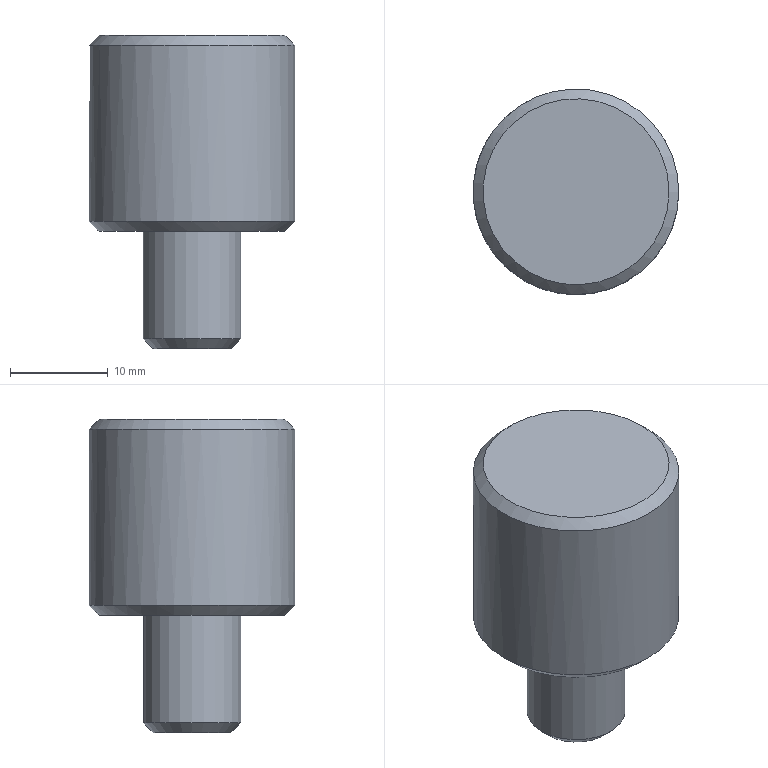Component | NX | FIXED_DOWEL_PIN | 1 solid | 8 faces | box 21 x 21 x 32 mm | volume 7791 mm3 | plane 3 | cone 3 | cylinder 2 | commonest cylinder face diameters 10 x1 21 x1
STEP:
#1=CARTESIAN_POINT('',(0.,0.,0.));
#2=DIRECTION('',(0.,0.,1.));
#3=DIRECTION('',(1.,0.,0.));
#4=AXIS2_PLACEMENT_3D('',#1,#2,#3);
#5=CARTESIAN_POINT('',(176.,0.,-79.));
#6=VERTEX_POINT('',#5);
#7=CARTESIAN_POINT('',(180.,0.,-79.));
#8=DIRECTION('',(0.,0.,-1.));
#9=DIRECTION('',(-1.,0.,0.));
#10=AXIS2_PLACEMENT_3D('',#7,#8,#9);
#11=CIRCLE('',#10,4.);
#12=CARTESIAN_POINT('',(180.,0.,-79.));
#13=DIRECTION('',(0.,0.,-1.));
#14=DIRECTION('',(-1.,0.,0.));
#15=AXIS2_PLACEMENT_3D('',#12,#13,#14);
#16=PLANE('',#15);
#17=CARTESIAN_POINT('',(0.,0.));
#18=DIRECTION('',(1.,0.));
#19=AXIS2_PLACEMENT_2D('',#17,#18);
#20=CIRCLE('',#19,4.);
#21=(GEOMETRIC_REPRESENTATION_CONTEXT(2)PARAMETRIC_REPRESENTATION_CONTEXT()REPRESENTATION_CONTEXT('',''));
#22=DEFINITIONAL_REPRESENTATION('',(#20),#21);
#23=PCURVE('',#16,#22);
#24=CARTESIAN_POINT('',(180.,0.,-78.));
#25=DIRECTION('',(0.,0.,1.));
#26=DIRECTION('',(1.,0.,0.));
#27=AXIS2_PLACEMENT_3D('',#24,#25,#26);
#28=CONICAL_SURFACE('',#27,5.,0.7854);
#29=CARTESIAN_POINT('',(9.425,-1.));
#30=DIRECTION('',(-1.,0.));
#31=VECTOR('',#30,1.);
#32=LINE('',#29,#31);
#33=(GEOMETRIC_REPRESENTATION_CONTEXT(2)PARAMETRIC_REPRESENTATION_CONTEXT()REPRESENTATION_CONTEXT('',''));
#34=DEFINITIONAL_REPRESENTATION('',(#32),#33);
#35=PCURVE('',#28,#34);
#36=SURFACE_CURVE('',#11,(#23,#35),.PCURVE_S1.);
#37=EDGE_CURVE('',#6,#6,#36,.T.);
#38=ORIENTED_EDGE('',*,*,#37,.T.);
#39=EDGE_LOOP('',(#38));
#40=FACE_BOUND('',#39,.T.);
#41=ADVANCED_FACE('',(#40),#16,.T.);
#42=CARTESIAN_POINT('',(175.,0.,-78.));
#43=VERTEX_POINT('',#42);
#44=CARTESIAN_POINT('',(180.,0.,-78.));
#45=DIRECTION('',(0.,0.,1.));
#46=DIRECTION('',(-1.,0.,0.));
#47=AXIS2_PLACEMENT_3D('',#44,#45,#46);
#48=CIRCLE('',#47,5.);
#49=CARTESIAN_POINT('',(180.,0.,-79.));
#50=DIRECTION('',(0.,0.,1.));
#51=DIRECTION('',(1.,0.,0.));
#52=AXIS2_PLACEMENT_3D('',#49,#50,#51);
#53=CYLINDRICAL_SURFACE('',#52,5.);
#54=CARTESIAN_POINT('',(3.142,1.));
#55=DIRECTION('',(1.,0.));
#56=VECTOR('',#55,1.);
#57=LINE('',#54,#56);
#58=(GEOMETRIC_REPRESENTATION_CONTEXT(2)PARAMETRIC_REPRESENTATION_CONTEXT()REPRESENTATION_CONTEXT('',''));
#59=DEFINITIONAL_REPRESENTATION('',(#57),#58);
#60=PCURVE('',#53,#59);
#61=CARTESIAN_POINT('',(3.142,0.));
#62=DIRECTION('',(1.,0.));
#63=VECTOR('',#62,1.);
#64=LINE('',#61,#63);
#65=(GEOMETRIC_REPRESENTATION_CONTEXT(2)PARAMETRIC_REPRESENTATION_CONTEXT()REPRESENTATION_CONTEXT('',''));
#66=DEFINITIONAL_REPRESENTATION('',(#64),#65);
#67=PCURVE('',#28,#66);
#68=SURFACE_CURVE('',#48,(#60,#67),.PCURVE_S1.);
#69=EDGE_CURVE('',#43,#43,#68,.T.);
#70=ORIENTED_EDGE('',*,*,#69,.T.);
#71=CARTESIAN_POINT('',(175.,0.,-67.));
#72=VERTEX_POINT('',#71);
#73=CARTESIAN_POINT('',(175.,0.,-78.));
#74=CARTESIAN_POINT('',(175.,0.,-67.));
#75=B_SPLINE_CURVE_WITH_KNOTS('',1,(#73,#74),.UNSPECIFIED.,.F.,.F.,(2,2),(1.,12.),.PIECEWISE_BEZIER_KNOTS.);
#76=CARTESIAN_POINT('',(9.425,0.));
#77=DIRECTION('',(0.,1.));
#78=VECTOR('',#77,1.);
#79=LINE('',#76,#78);
#80=(GEOMETRIC_REPRESENTATION_CONTEXT(2)PARAMETRIC_REPRESENTATION_CONTEXT()REPRESENTATION_CONTEXT('',''));
#81=DEFINITIONAL_REPRESENTATION('',(#79),#80);
#82=PCURVE('',#53,#81);
#83=CARTESIAN_POINT('',(3.142,0.));
#84=DIRECTION('',(0.,1.));
#85=VECTOR('',#84,1.);
#86=LINE('',#83,#85);
#87=(GEOMETRIC_REPRESENTATION_CONTEXT(2)PARAMETRIC_REPRESENTATION_CONTEXT()REPRESENTATION_CONTEXT('',''));
#88=DEFINITIONAL_REPRESENTATION('',(#86),#87);
#89=PCURVE('',#53,#88);
#90=SEAM_CURVE('',#75,(#82,#89),.PCURVE_S1.);
#91=EDGE_CURVE('',#43,#72,#90,.T.);
#92=ORIENTED_EDGE('',*,*,#91,.T.);
#93=CARTESIAN_POINT('',(180.,0.,-67.));
#94=DIRECTION('',(0.,0.,1.));
#95=DIRECTION('',(-1.,0.,0.));
#96=AXIS2_PLACEMENT_3D('',#93,#94,#95);
#97=CIRCLE('',#96,5.);
#98=CARTESIAN_POINT('',(3.142,12.));
#99=DIRECTION('',(1.,0.));
#100=VECTOR('',#99,1.);
#101=LINE('',#98,#100);
#102=(GEOMETRIC_REPRESENTATION_CONTEXT(2)PARAMETRIC_REPRESENTATION_CONTEXT()REPRESENTATION_CONTEXT('',''));
#103=DEFINITIONAL_REPRESENTATION('',(#101),#102);
#104=PCURVE('',#53,#103);
#105=CARTESIAN_POINT('',(180.,0.,-67.));
#106=DIRECTION('',(0.,0.,-1.));
#107=DIRECTION('',(-1.,0.,0.));
#108=AXIS2_PLACEMENT_3D('',#105,#106,#107);
#109=PLANE('',#108);
#110=CARTESIAN_POINT('',(5.,0.));
#111=CARTESIAN_POINT('',(5.,-8.66));
#112=CARTESIAN_POINT('',(-2.5,-4.33));
#113=CARTESIAN_POINT('',(-10.,-0.));
#114=CARTESIAN_POINT('',(-2.5,4.33));
#115=CARTESIAN_POINT('',(5.,8.66));
#116=CARTESIAN_POINT('',(5.,0.));
#117=(BOUNDED_CURVE()B_SPLINE_CURVE(2,(#110,#111,#112,#113,#114,#115,#116),.UNSPECIFIED.,.T.,.F.)B_SPLINE_CURVE_WITH_KNOTS((1,2,2,2,2,1),(-2.094,0.,2.094,4.189,6.283,8.378),.UNSPECIFIED.)CURVE()GEOMETRIC_REPRESENTATION_ITEM()RATIONAL_B_SPLINE_CURVE((1.,0.5,1.,0.5,1.,0.5,1.))REPRESENTATION_ITEM(''));
#118=(GEOMETRIC_REPRESENTATION_CONTEXT(2)PARAMETRIC_REPRESENTATION_CONTEXT()REPRESENTATION_CONTEXT('',''));
#119=DEFINITIONAL_REPRESENTATION('',(#117),#118);
#120=PCURVE('',#109,#119);
#121=SURFACE_CURVE('',#97,(#104,#120),.PCURVE_S1.);
#122=EDGE_CURVE('',#72,#72,#121,.T.);
#123=ORIENTED_EDGE('',*,*,#122,.F.);
#124=ORIENTED_EDGE('',*,*,#91,.F.);
#125=EDGE_LOOP('',(#70,#92,#123,#124));
#126=FACE_BOUND('',#125,.T.);
#127=ADVANCED_FACE('',(#126),#53,.T.);
#128=CARTESIAN_POINT('',(189.5,0.,-47.));
#129=VERTEX_POINT('',#128);
#130=CARTESIAN_POINT('',(180.,0.,-47.));
#131=DIRECTION('',(0.,0.,1.));
#132=DIRECTION('',(1.,0.,0.));
#133=AXIS2_PLACEMENT_3D('',#130,#131,#132);
#134=CIRCLE('',#133,9.5);
#135=CARTESIAN_POINT('',(180.,0.,-47.));
#136=DIRECTION('',(0.,0.,1.));
#137=DIRECTION('',(1.,0.,0.));
#138=AXIS2_PLACEMENT_3D('',#135,#136,#137);
#139=PLANE('',#138);
#140=CARTESIAN_POINT('',(0.,0.));
#141=DIRECTION('',(1.,0.));
#142=AXIS2_PLACEMENT_2D('',#140,#141);
#143=CIRCLE('',#142,9.5);
#144=(GEOMETRIC_REPRESENTATION_CONTEXT(2)PARAMETRIC_REPRESENTATION_CONTEXT()REPRESENTATION_CONTEXT('',''));
#145=DEFINITIONAL_REPRESENTATION('',(#143),#144);
#146=PCURVE('',#139,#145);
#147=CARTESIAN_POINT('',(180.,0.,-48.));
#148=DIRECTION('',(0.,0.,-1.));
#149=DIRECTION('',(-1.,0.,0.));
#150=AXIS2_PLACEMENT_3D('',#147,#148,#149);
#151=CONICAL_SURFACE('',#150,10.5,0.7854);
#152=CARTESIAN_POINT('',(9.425,-1.));
#153=DIRECTION('',(-1.,0.));
#154=VECTOR('',#153,1.);
#155=LINE('',#152,#154);
#156=(GEOMETRIC_REPRESENTATION_CONTEXT(2)PARAMETRIC_REPRESENTATION_CONTEXT()REPRESENTATION_CONTEXT('',''));
#157=DEFINITIONAL_REPRESENTATION('',(#155),#156);
#158=PCURVE('',#151,#157);
#159=SURFACE_CURVE('',#134,(#146,#158),.PCURVE_S1.);
#160=EDGE_CURVE('',#129,#129,#159,.T.);
#161=ORIENTED_EDGE('',*,*,#160,.T.);
#162=EDGE_LOOP('',(#161));
#163=FACE_BOUND('',#162,.T.);
#164=ADVANCED_FACE('',(#163),#139,.T.);
#165=CARTESIAN_POINT('',(170.5,0.,-67.));
#166=VERTEX_POINT('',#165);
#167=CARTESIAN_POINT('',(180.,0.,-67.));
#168=DIRECTION('',(0.,0.,-1.));
#169=DIRECTION('',(-1.,0.,0.));
#170=AXIS2_PLACEMENT_3D('',#167,#168,#169);
#171=CIRCLE('',#170,9.5);
#172=CARTESIAN_POINT('',(0.,0.));
#173=DIRECTION('',(1.,0.));
#174=AXIS2_PLACEMENT_2D('',#172,#173);
#175=CIRCLE('',#174,9.5);
#176=(GEOMETRIC_REPRESENTATION_CONTEXT(2)PARAMETRIC_REPRESENTATION_CONTEXT()REPRESENTATION_CONTEXT('',''));
#177=DEFINITIONAL_REPRESENTATION('',(#175),#176);
#178=PCURVE('',#109,#177);
#179=CARTESIAN_POINT('',(180.,0.,-66.));
#180=DIRECTION('',(0.,0.,1.));
#181=DIRECTION('',(1.,0.,0.));
#182=AXIS2_PLACEMENT_3D('',#179,#180,#181);
#183=CONICAL_SURFACE('',#182,10.5,0.7854);
#184=CARTESIAN_POINT('',(9.425,-1.));
#185=DIRECTION('',(-1.,0.));
#186=VECTOR('',#185,1.);
#187=LINE('',#184,#186);
#188=(GEOMETRIC_REPRESENTATION_CONTEXT(2)PARAMETRIC_REPRESENTATION_CONTEXT()REPRESENTATION_CONTEXT('',''));
#189=DEFINITIONAL_REPRESENTATION('',(#187),#188);
#190=PCURVE('',#183,#189);
#191=SURFACE_CURVE('',#171,(#178,#190),.PCURVE_S1.);
#192=EDGE_CURVE('',#166,#166,#191,.T.);
#193=ORIENTED_EDGE('',*,*,#192,.T.);
#194=EDGE_LOOP('',(#193));
#195=FACE_BOUND('',#194,.T.);
#196=ORIENTED_EDGE('',*,*,#122,.T.);
#197=EDGE_LOOP('',(#196));
#198=FACE_BOUND('',#197,.T.);
#199=ADVANCED_FACE('',(#195,#198),#109,.T.);
#200=CARTESIAN_POINT('',(169.5,0.,-66.));
#201=VERTEX_POINT('',#200);
#202=CARTESIAN_POINT('',(190.5,-0.,-66.));
#203=VERTEX_POINT('',#202);
#204=CARTESIAN_POINT('',(180.,0.,-66.));
#205=DIRECTION('',(0.,0.,1.));
#206=DIRECTION('',(-1.,0.,0.));
#207=AXIS2_PLACEMENT_3D('',#204,#205,#206);
#208=CIRCLE('',#207,10.5);
#209=CARTESIAN_POINT('',(180.,0.,-67.));
#210=DIRECTION('',(0.,0.,1.));
#211=DIRECTION('',(1.,0.,0.));
#212=AXIS2_PLACEMENT_3D('',#209,#210,#211);
#213=CYLINDRICAL_SURFACE('',#212,10.5);
#214=CARTESIAN_POINT('',(3.142,1.));
#215=DIRECTION('',(1.,0.));
#216=VECTOR('',#215,1.);
#217=LINE('',#214,#216);
#218=(GEOMETRIC_REPRESENTATION_CONTEXT(2)PARAMETRIC_REPRESENTATION_CONTEXT()REPRESENTATION_CONTEXT('',''));
#219=DEFINITIONAL_REPRESENTATION('',(#217),#218);
#220=PCURVE('',#213,#219);
#221=CARTESIAN_POINT('',(3.142,0.));
#222=DIRECTION('',(1.,0.));
#223=VECTOR('',#222,1.);
#224=LINE('',#221,#223);
#225=(GEOMETRIC_REPRESENTATION_CONTEXT(2)PARAMETRIC_REPRESENTATION_CONTEXT()REPRESENTATION_CONTEXT('',''));
#226=DEFINITIONAL_REPRESENTATION('',(#224),#225);
#227=PCURVE('',#183,#226);
#228=SURFACE_CURVE('',#208,(#220,#227),.PCURVE_S1.);
#229=EDGE_CURVE('',#201,#203,#228,.T.);
#230=ORIENTED_EDGE('',*,*,#229,.T.);
#231=CARTESIAN_POINT('',(190.5,0.,-48.));
#232=VERTEX_POINT('',#231);
#233=CARTESIAN_POINT('',(190.5,0.,-66.));
#234=CARTESIAN_POINT('',(190.5,0.,-48.));
#235=B_SPLINE_CURVE_WITH_KNOTS('',1,(#233,#234),.UNSPECIFIED.,.F.,.F.,(2,2),(1.,19.),.PIECEWISE_BEZIER_KNOTS.);
#236=CARTESIAN_POINT('',(6.283,0.));
#237=DIRECTION('',(0.,1.));
#238=VECTOR('',#237,1.);
#239=LINE('',#236,#238);
#240=(GEOMETRIC_REPRESENTATION_CONTEXT(2)PARAMETRIC_REPRESENTATION_CONTEXT()REPRESENTATION_CONTEXT('',''));
#241=DEFINITIONAL_REPRESENTATION('',(#239),#240);
#242=PCURVE('',#213,#241);
#243=CARTESIAN_POINT('',(0.,0.));
#244=DIRECTION('',(0.,1.));
#245=VECTOR('',#244,1.);
#246=LINE('',#243,#245);
#247=(GEOMETRIC_REPRESENTATION_CONTEXT(2)PARAMETRIC_REPRESENTATION_CONTEXT()REPRESENTATION_CONTEXT('',''));
#248=DEFINITIONAL_REPRESENTATION('',(#246),#247);
#249=PCURVE('',#213,#248);
#250=SEAM_CURVE('',#235,(#242,#249),.PCURVE_S1.);
#251=EDGE_CURVE('',#203,#232,#250,.T.);
#252=ORIENTED_EDGE('',*,*,#251,.T.);
#253=CARTESIAN_POINT('',(180.,0.,-48.));
#254=DIRECTION('',(0.,0.,-1.));
#255=DIRECTION('',(1.,0.,0.));
#256=AXIS2_PLACEMENT_3D('',#253,#254,#255);
#257=CIRCLE('',#256,10.5);
#258=CARTESIAN_POINT('',(6.283,19.));
#259=DIRECTION('',(-1.,0.));
#260=VECTOR('',#259,1.);
#261=LINE('',#258,#260);
#262=(GEOMETRIC_REPRESENTATION_CONTEXT(2)PARAMETRIC_REPRESENTATION_CONTEXT()REPRESENTATION_CONTEXT('',''));
#263=DEFINITIONAL_REPRESENTATION('',(#261),#262);
#264=PCURVE('',#213,#263);
#265=CARTESIAN_POINT('',(3.142,0.));
#266=DIRECTION('',(1.,0.));
#267=VECTOR('',#266,1.);
#268=LINE('',#265,#267);
#269=(GEOMETRIC_REPRESENTATION_CONTEXT(2)PARAMETRIC_REPRESENTATION_CONTEXT()REPRESENTATION_CONTEXT('',''));
#270=DEFINITIONAL_REPRESENTATION('',(#268),#269);
#271=PCURVE('',#151,#270);
#272=SURFACE_CURVE('',#257,(#264,#271),.PCURVE_S1.);
#273=EDGE_CURVE('',#232,#232,#272,.T.);
#274=ORIENTED_EDGE('',*,*,#273,.T.);
#275=ORIENTED_EDGE('',*,*,#251,.F.);
#276=CARTESIAN_POINT('',(180.,0.,-66.));
#277=DIRECTION('',(0.,0.,1.));
#278=DIRECTION('',(-1.,0.,0.));
#279=AXIS2_PLACEMENT_3D('',#276,#277,#278);
#280=CIRCLE('',#279,10.5);
#281=CARTESIAN_POINT('',(-3.142,1.));
#282=DIRECTION('',(1.,0.));
#283=VECTOR('',#282,1.);
#284=LINE('',#281,#283);
#285=(GEOMETRIC_REPRESENTATION_CONTEXT(2)PARAMETRIC_REPRESENTATION_CONTEXT()REPRESENTATION_CONTEXT('',''));
#286=DEFINITIONAL_REPRESENTATION('',(#284),#285);
#287=PCURVE('',#213,#286);
#288=CARTESIAN_POINT('',(3.142,0.));
#289=DIRECTION('',(1.,0.));
#290=VECTOR('',#289,1.);
#291=LINE('',#288,#290);
#292=(GEOMETRIC_REPRESENTATION_CONTEXT(2)PARAMETRIC_REPRESENTATION_CONTEXT()REPRESENTATION_CONTEXT('',''));
#293=DEFINITIONAL_REPRESENTATION('',(#291),#292);
#294=PCURVE('',#183,#293);
#295=SURFACE_CURVE('',#280,(#287,#294),.PCURVE_S1.);
#296=EDGE_CURVE('',#203,#201,#295,.T.);
#297=ORIENTED_EDGE('',*,*,#296,.T.);
#298=EDGE_LOOP('',(#230,#252,#274,#275,#297));
#299=FACE_BOUND('',#298,.T.);
#300=ADVANCED_FACE('',(#299),#213,.T.);
#301=ORIENTED_EDGE('',*,*,#37,.F.);
#302=CARTESIAN_POINT('',(176.,0.,-79.));
#303=CARTESIAN_POINT('',(175.,0.,-78.));
#304=B_SPLINE_CURVE_WITH_KNOTS('',1,(#302,#303),.UNSPECIFIED.,.F.,.F.,(2,2),(-1.414,0.),.PIECEWISE_BEZIER_KNOTS.);
#305=CARTESIAN_POINT('',(9.425,0.));
#306=DIRECTION('',(0.,1.));
#307=VECTOR('',#306,1.);
#308=LINE('',#305,#307);
#309=(GEOMETRIC_REPRESENTATION_CONTEXT(2)PARAMETRIC_REPRESENTATION_CONTEXT()REPRESENTATION_CONTEXT('',''));
#310=DEFINITIONAL_REPRESENTATION('',(#308),#309);
#311=PCURVE('',#28,#310);
#312=CARTESIAN_POINT('',(3.142,0.));
#313=DIRECTION('',(0.,1.));
#314=VECTOR('',#313,1.);
#315=LINE('',#312,#314);
#316=(GEOMETRIC_REPRESENTATION_CONTEXT(2)PARAMETRIC_REPRESENTATION_CONTEXT()REPRESENTATION_CONTEXT('',''));
#317=DEFINITIONAL_REPRESENTATION('',(#315),#316);
#318=PCURVE('',#28,#317);
#319=SEAM_CURVE('',#304,(#311,#318),.PCURVE_S1.);
#320=EDGE_CURVE('',#6,#43,#319,.T.);
#321=ORIENTED_EDGE('',*,*,#320,.T.);
#322=ORIENTED_EDGE('',*,*,#69,.F.);
#323=ORIENTED_EDGE('',*,*,#320,.F.);
#324=EDGE_LOOP('',(#301,#321,#322,#323));
#325=FACE_BOUND('',#324,.T.);
#326=ADVANCED_FACE('',(#325),#28,.T.);
#327=ORIENTED_EDGE('',*,*,#192,.F.);
#328=CARTESIAN_POINT('',(170.5,0.,-67.));
#329=CARTESIAN_POINT('',(169.5,0.,-66.));
#330=B_SPLINE_CURVE_WITH_KNOTS('',1,(#328,#329),.UNSPECIFIED.,.F.,.F.,(2,2),(-1.414,0.),.PIECEWISE_BEZIER_KNOTS.);
#331=CARTESIAN_POINT('',(9.425,0.));
#332=DIRECTION('',(0.,1.));
#333=VECTOR('',#332,1.);
#334=LINE('',#331,#333);
#335=(GEOMETRIC_REPRESENTATION_CONTEXT(2)PARAMETRIC_REPRESENTATION_CONTEXT()REPRESENTATION_CONTEXT('',''));
#336=DEFINITIONAL_REPRESENTATION('',(#334),#335);
#337=PCURVE('',#183,#336);
#338=CARTESIAN_POINT('',(3.142,0.));
#339=DIRECTION('',(0.,1.));
#340=VECTOR('',#339,1.);
#341=LINE('',#338,#340);
#342=(GEOMETRIC_REPRESENTATION_CONTEXT(2)PARAMETRIC_REPRESENTATION_CONTEXT()REPRESENTATION_CONTEXT('',''));
#343=DEFINITIONAL_REPRESENTATION('',(#341),#342);
#344=PCURVE('',#183,#343);
#345=SEAM_CURVE('',#330,(#337,#344),.PCURVE_S1.);
#346=EDGE_CURVE('',#166,#201,#345,.T.);
#347=ORIENTED_EDGE('',*,*,#346,.T.);
#348=ORIENTED_EDGE('',*,*,#296,.F.);
#349=ORIENTED_EDGE('',*,*,#229,.F.);
#350=ORIENTED_EDGE('',*,*,#346,.F.);
#351=EDGE_LOOP('',(#327,#347,#348,#349,#350));
#352=FACE_BOUND('',#351,.T.);
#353=ADVANCED_FACE('',(#352),#183,.T.);
#354=ORIENTED_EDGE('',*,*,#160,.F.);
#355=CARTESIAN_POINT('',(189.5,0.,-47.));
#356=CARTESIAN_POINT('',(190.5,0.,-48.));
#357=B_SPLINE_CURVE_WITH_KNOTS('',1,(#355,#356),.UNSPECIFIED.,.F.,.F.,(2,2),(-1.414,0.),.PIECEWISE_BEZIER_KNOTS.);
#358=CARTESIAN_POINT('',(9.425,0.));
#359=DIRECTION('',(0.,1.));
#360=VECTOR('',#359,1.);
#361=LINE('',#358,#360);
#362=(GEOMETRIC_REPRESENTATION_CONTEXT(2)PARAMETRIC_REPRESENTATION_CONTEXT()REPRESENTATION_CONTEXT('',''));
#363=DEFINITIONAL_REPRESENTATION('',(#361),#362);
#364=PCURVE('',#151,#363);
#365=CARTESIAN_POINT('',(3.142,0.));
#366=DIRECTION('',(0.,1.));
#367=VECTOR('',#366,1.);
#368=LINE('',#365,#367);
#369=(GEOMETRIC_REPRESENTATION_CONTEXT(2)PARAMETRIC_REPRESENTATION_CONTEXT()REPRESENTATION_CONTEXT('',''));
#370=DEFINITIONAL_REPRESENTATION('',(#368),#369);
#371=PCURVE('',#151,#370);
#372=SEAM_CURVE('',#357,(#364,#371),.PCURVE_S1.);
#373=EDGE_CURVE('',#129,#232,#372,.T.);
#374=ORIENTED_EDGE('',*,*,#373,.T.);
#375=ORIENTED_EDGE('',*,*,#273,.F.);
#376=ORIENTED_EDGE('',*,*,#373,.F.);
#377=EDGE_LOOP('',(#354,#374,#375,#376));
#378=FACE_BOUND('',#377,.T.);
#379=ADVANCED_FACE('',(#378),#151,.T.);
#380=CLOSED_SHELL('',(#41,#127,#164,#199,#300,#326,#353,#379));
#381=MANIFOLD_SOLID_BREP('',#380);
#382=(LENGTH_UNIT()NAMED_UNIT(*)SI_UNIT(.MILLI.,.METRE.));
#383=UNCERTAINTY_MEASURE_WITH_UNIT(LENGTH_MEASURE(0.00001),#382,'','');
#384=(NAMED_UNIT(*)PLANE_ANGLE_UNIT()SI_UNIT($,.RADIAN.));
#385=(NAMED_UNIT(*)SI_UNIT($,.STERADIAN.)SOLID_ANGLE_UNIT());
#386=(GEOMETRIC_REPRESENTATION_CONTEXT(3)GLOBAL_UNCERTAINTY_ASSIGNED_CONTEXT((#383))GLOBAL_UNIT_ASSIGNED_CONTEXT((#382,#384,#385))REPRESENTATION_CONTEXT('',''));
#387=ADVANCED_BREP_SHAPE_REPRESENTATION('',(#4,#381),#386);